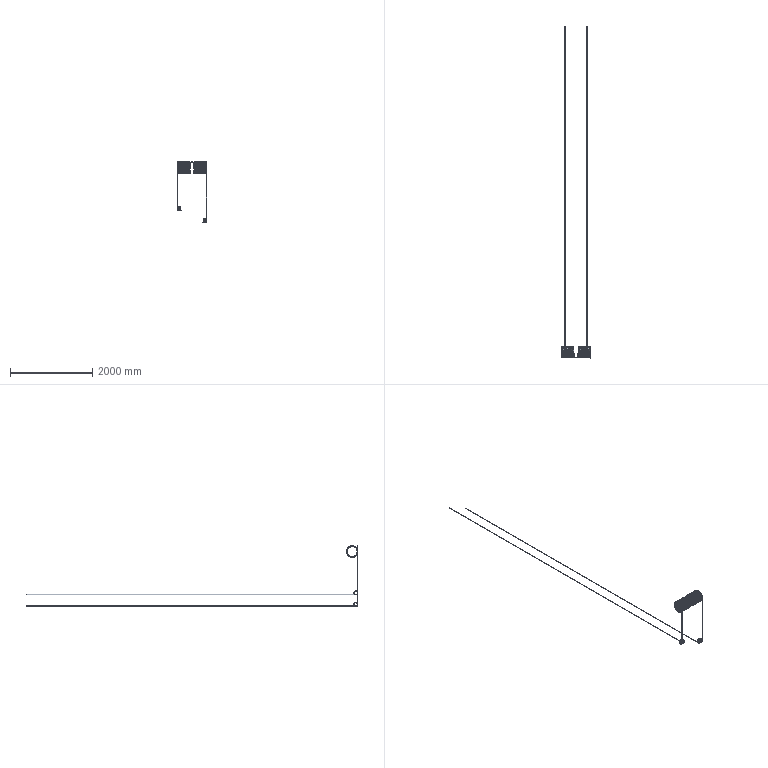Component | SolidWorks | LiftingAndOperatingMechanism-1_28-1 | 2 solids | 34 faces | volume 4359504 mm3 | plane 14 | spline 12 | cylinder 8 | commonest cylinder face diameters 10 x8